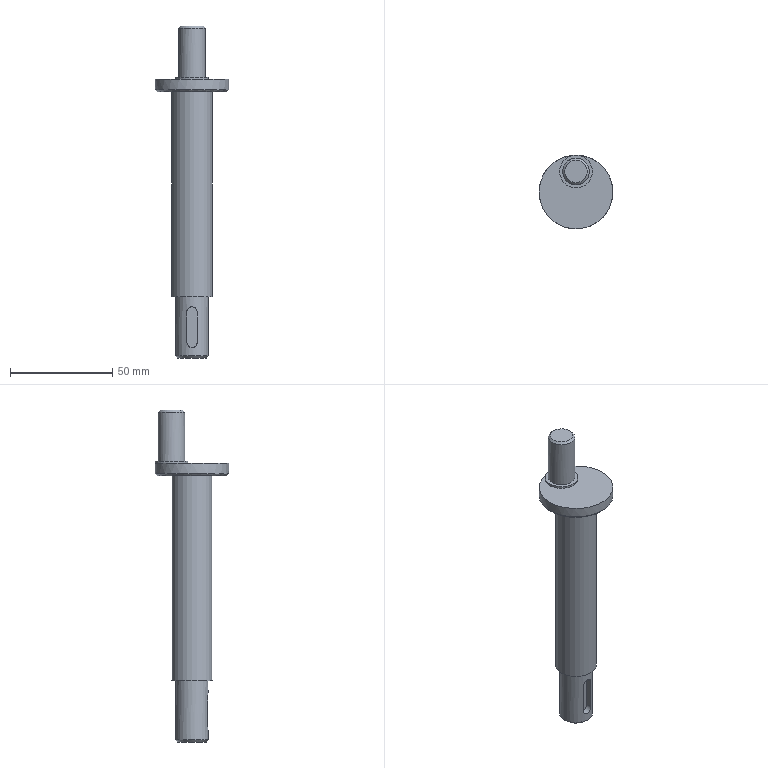Component | NX | 10_CRANKSHAFT | 5 solids | 23 faces | volume 46703 mm3 | plane 13 | cylinder 7 | cone 3 | commonest cylinder face diameters 16 x2 5 x2 13 x1 36 x1 20 x1